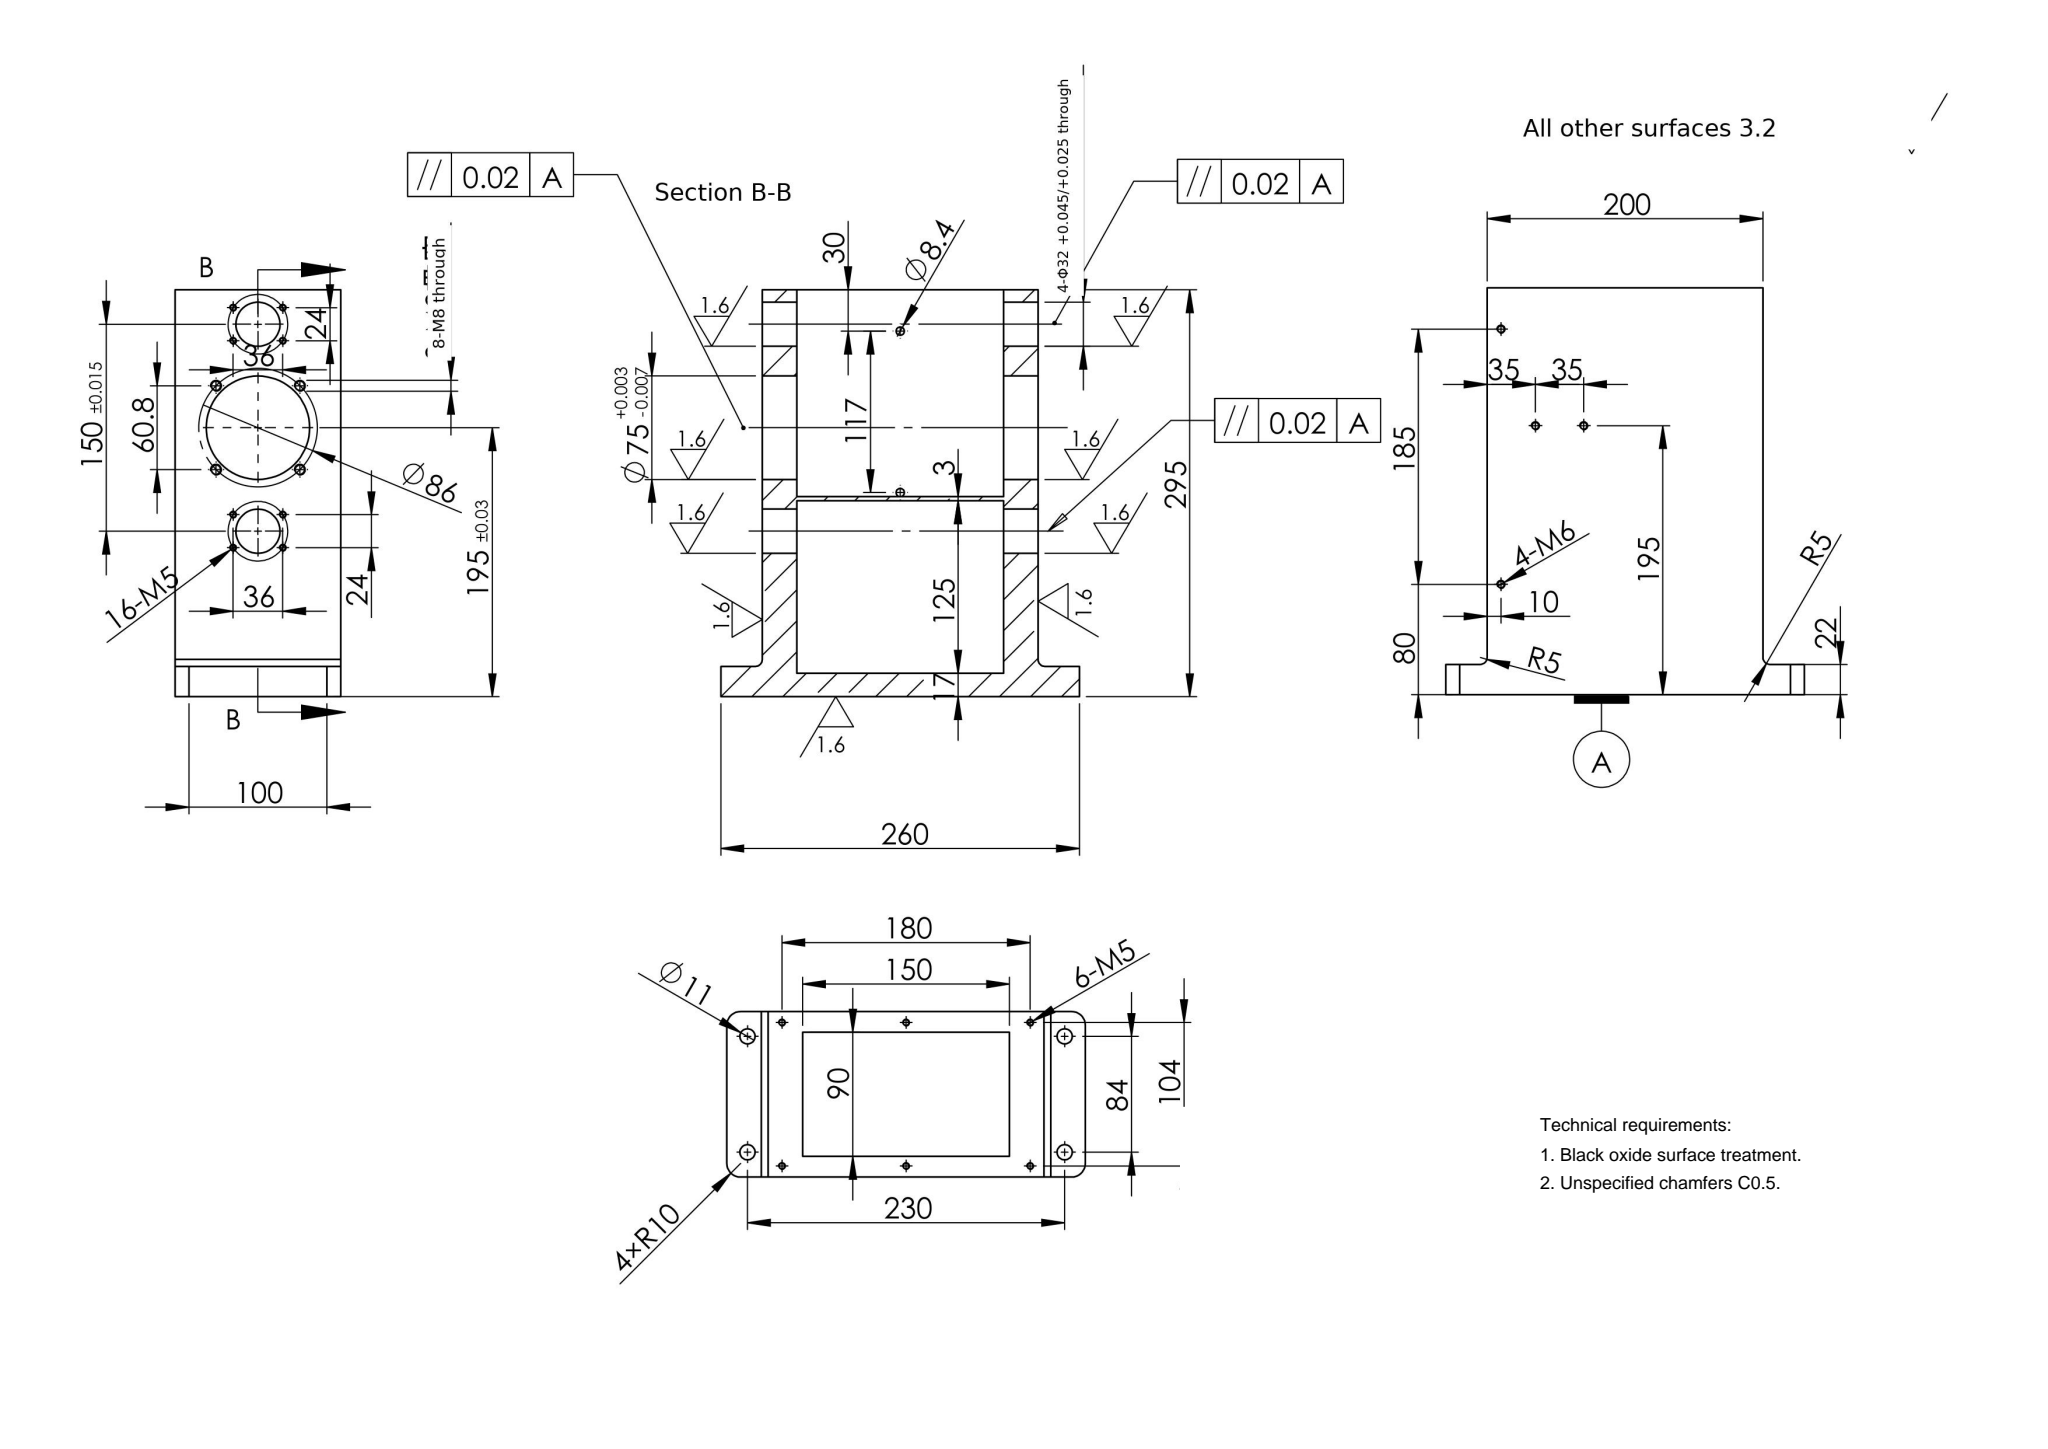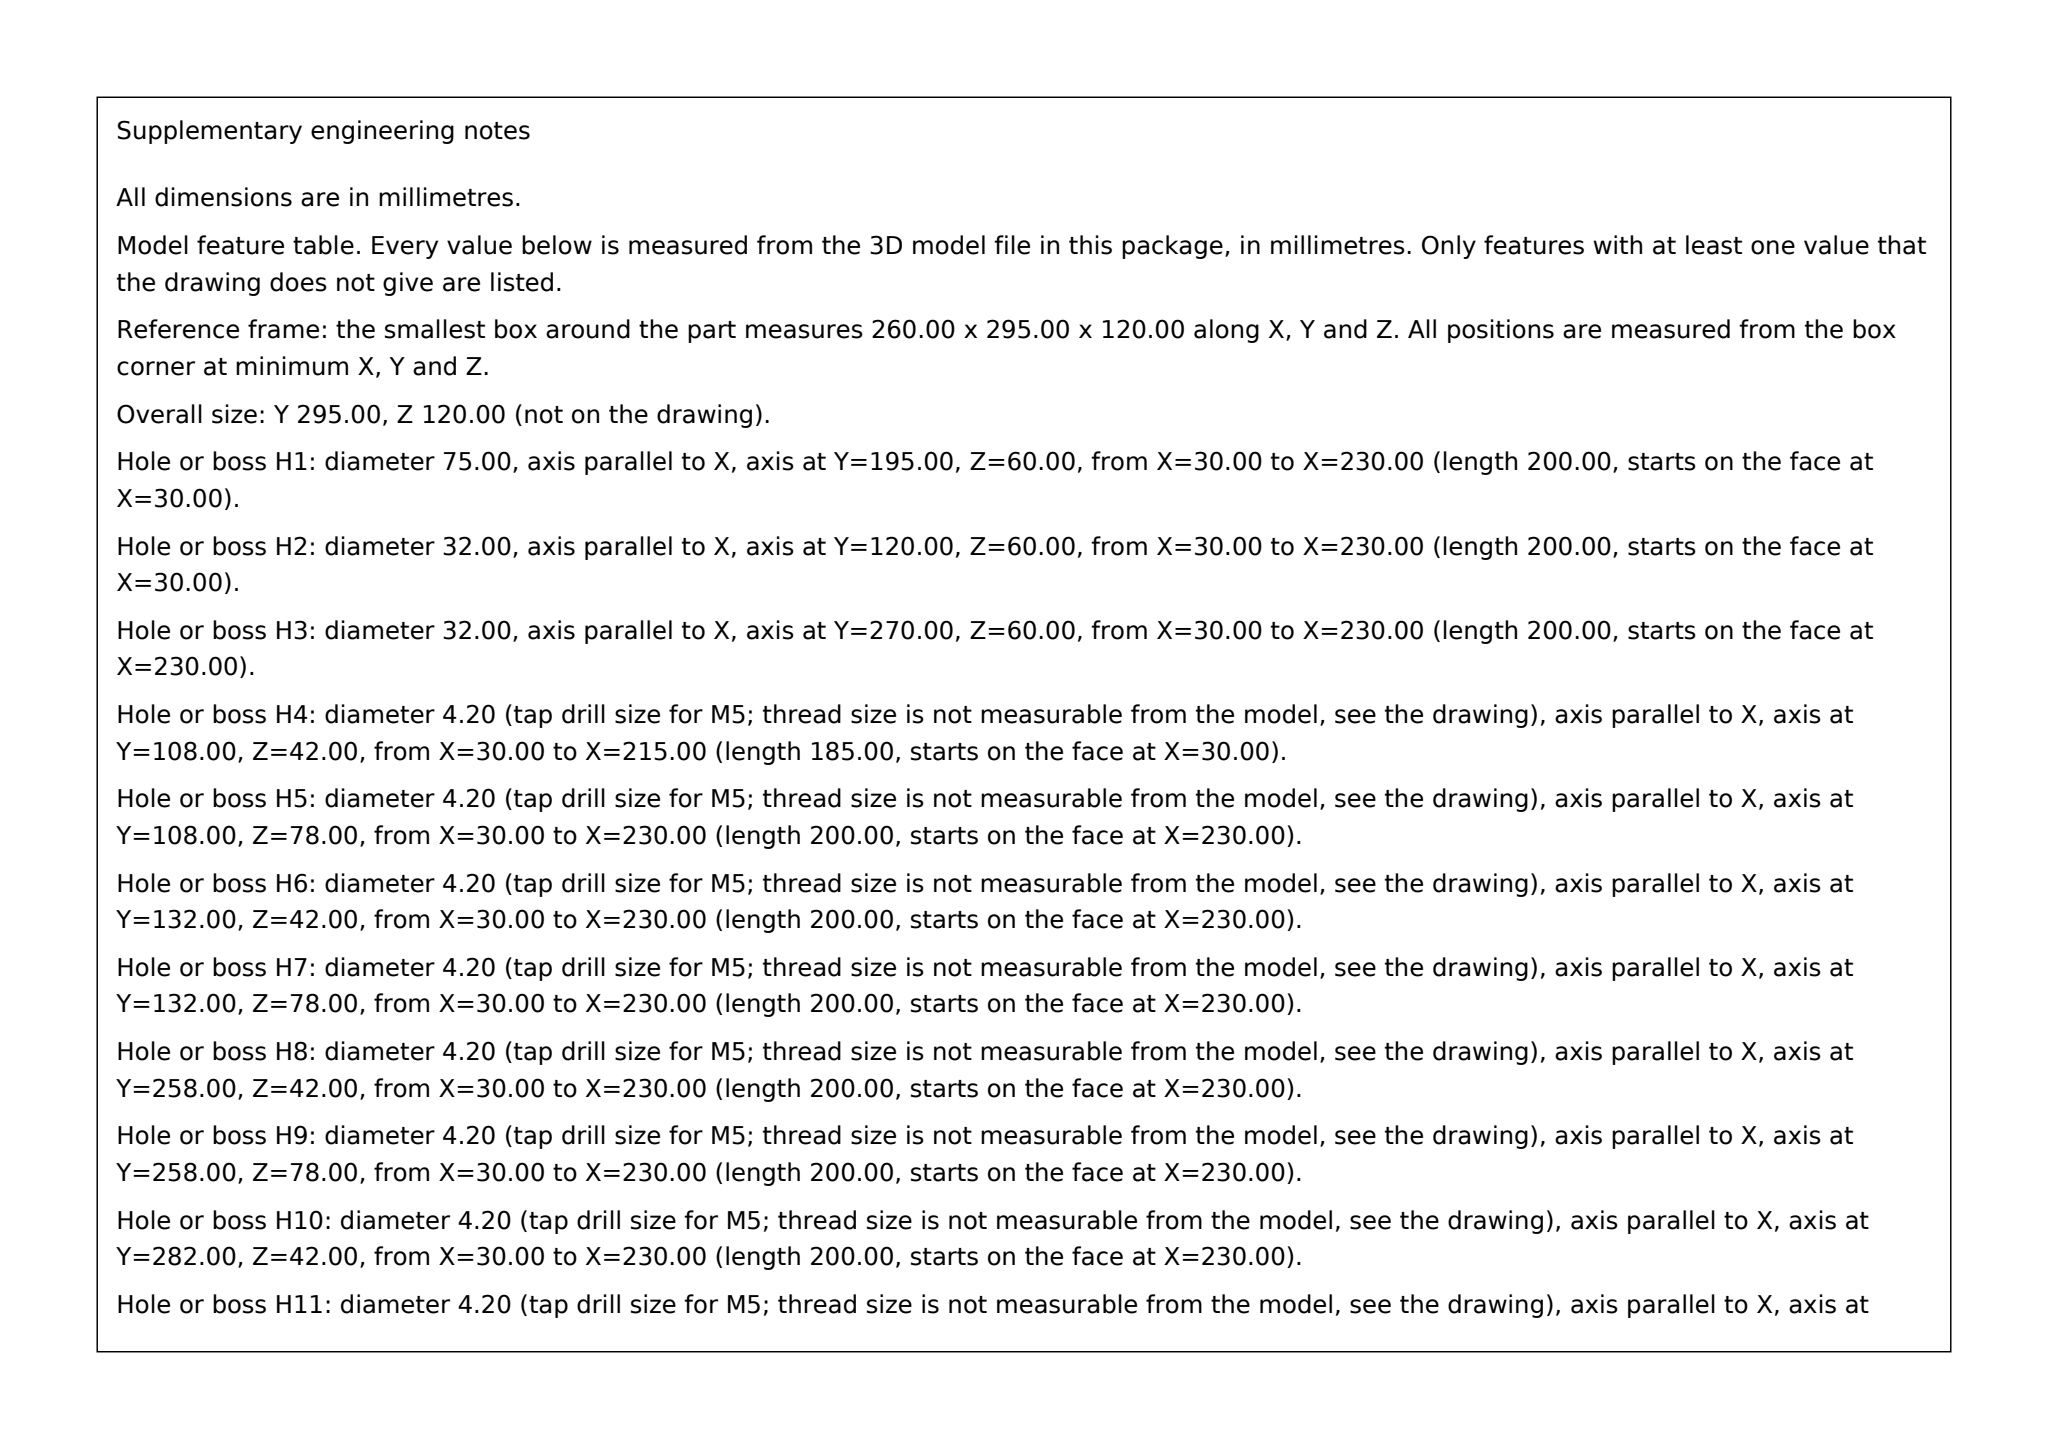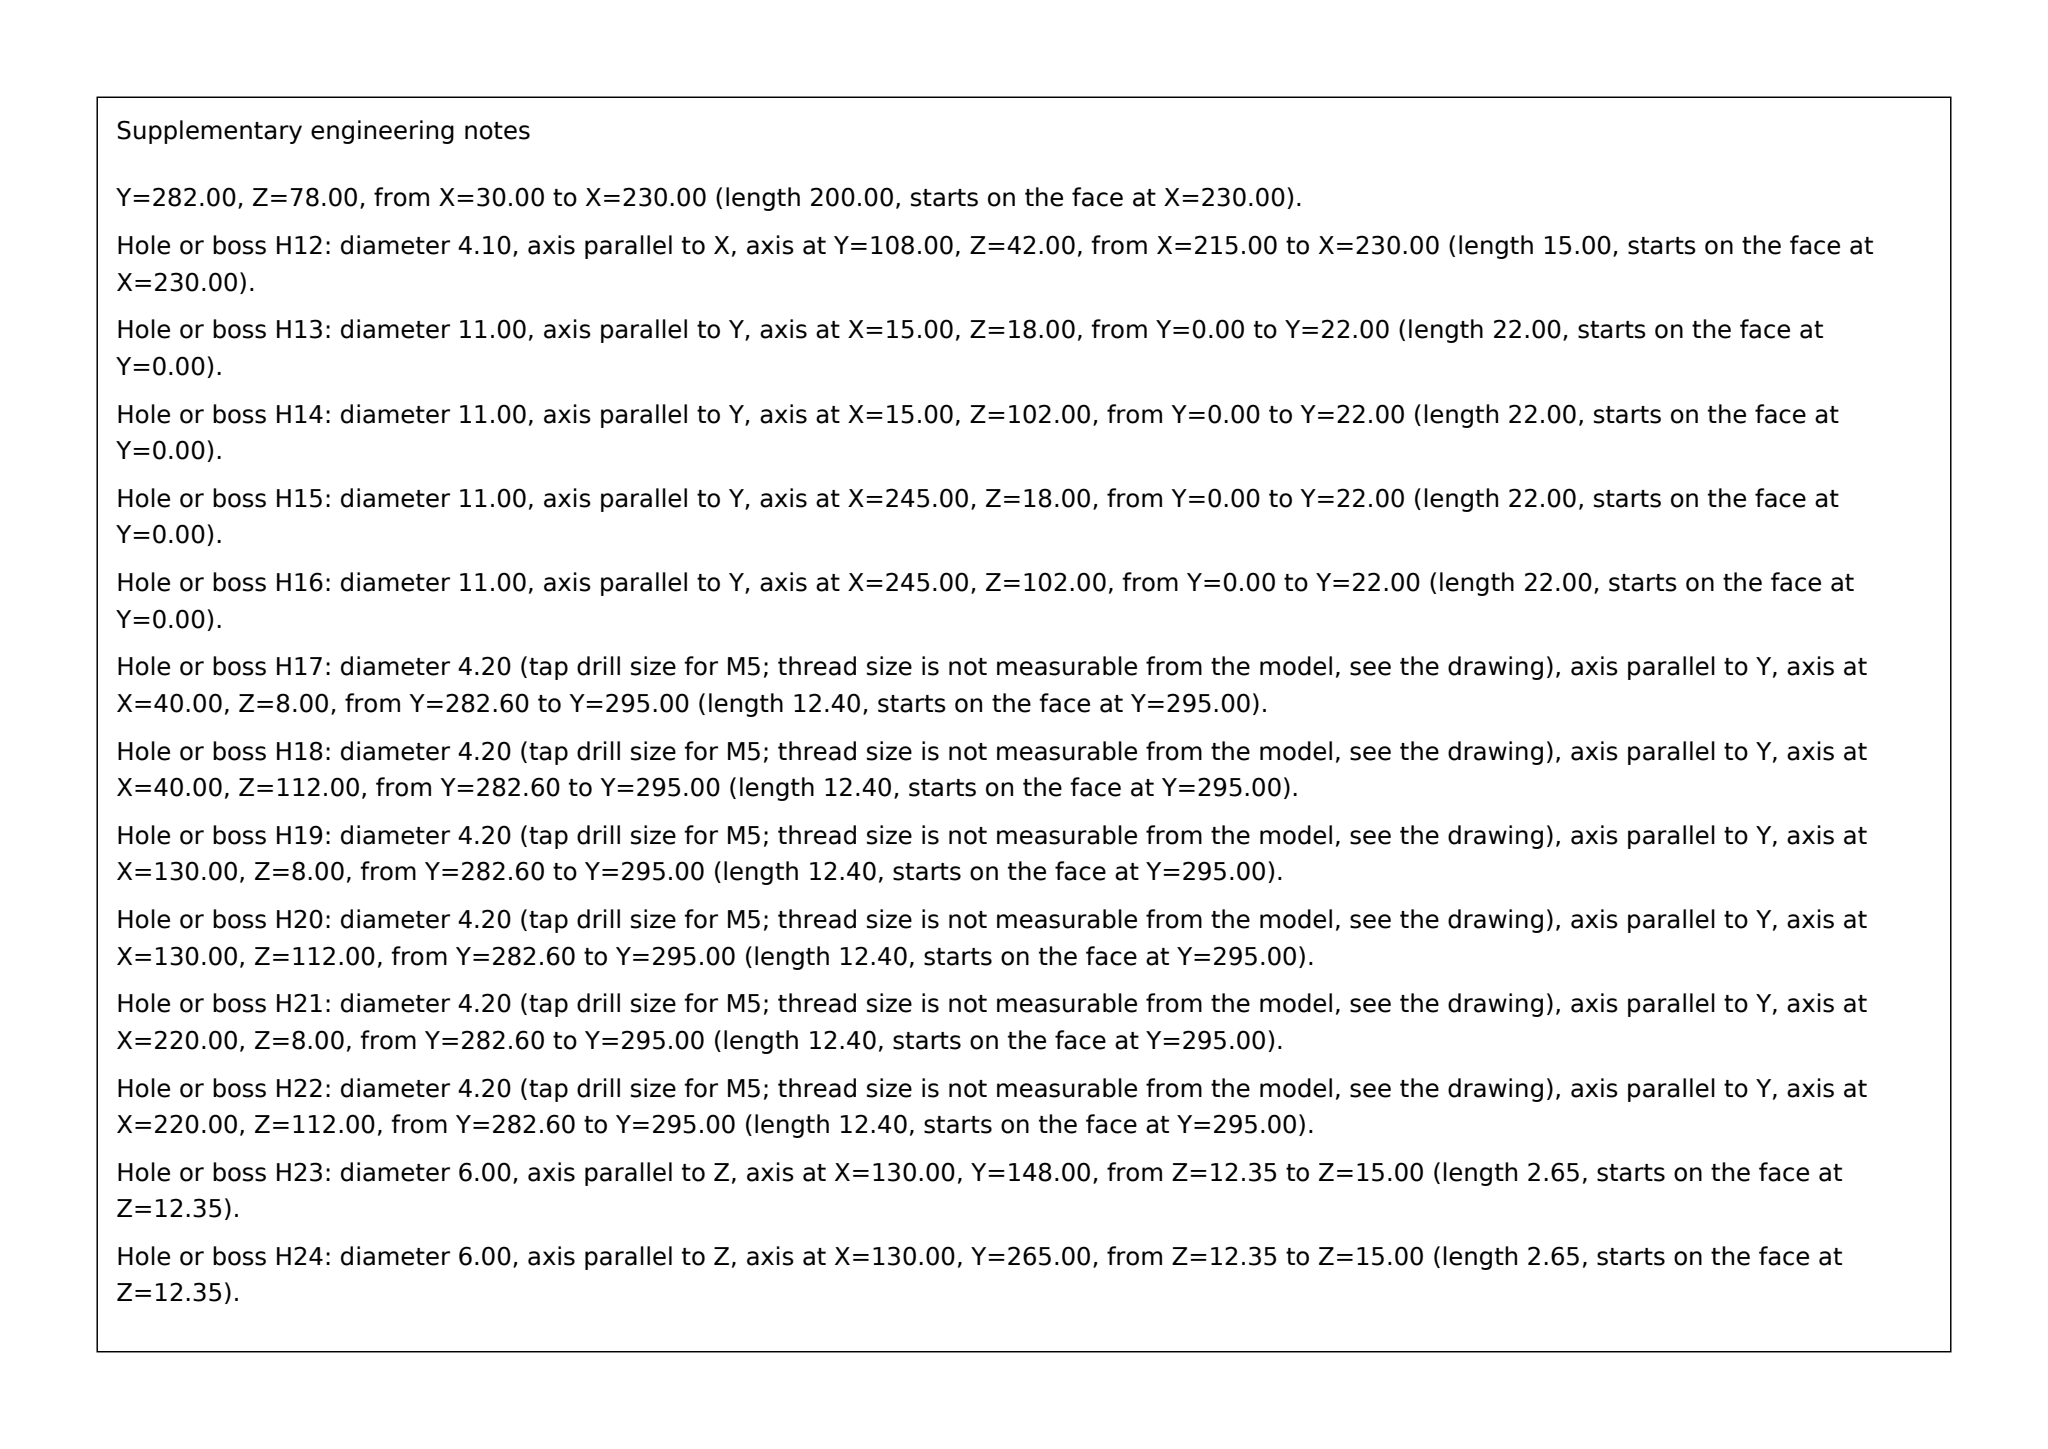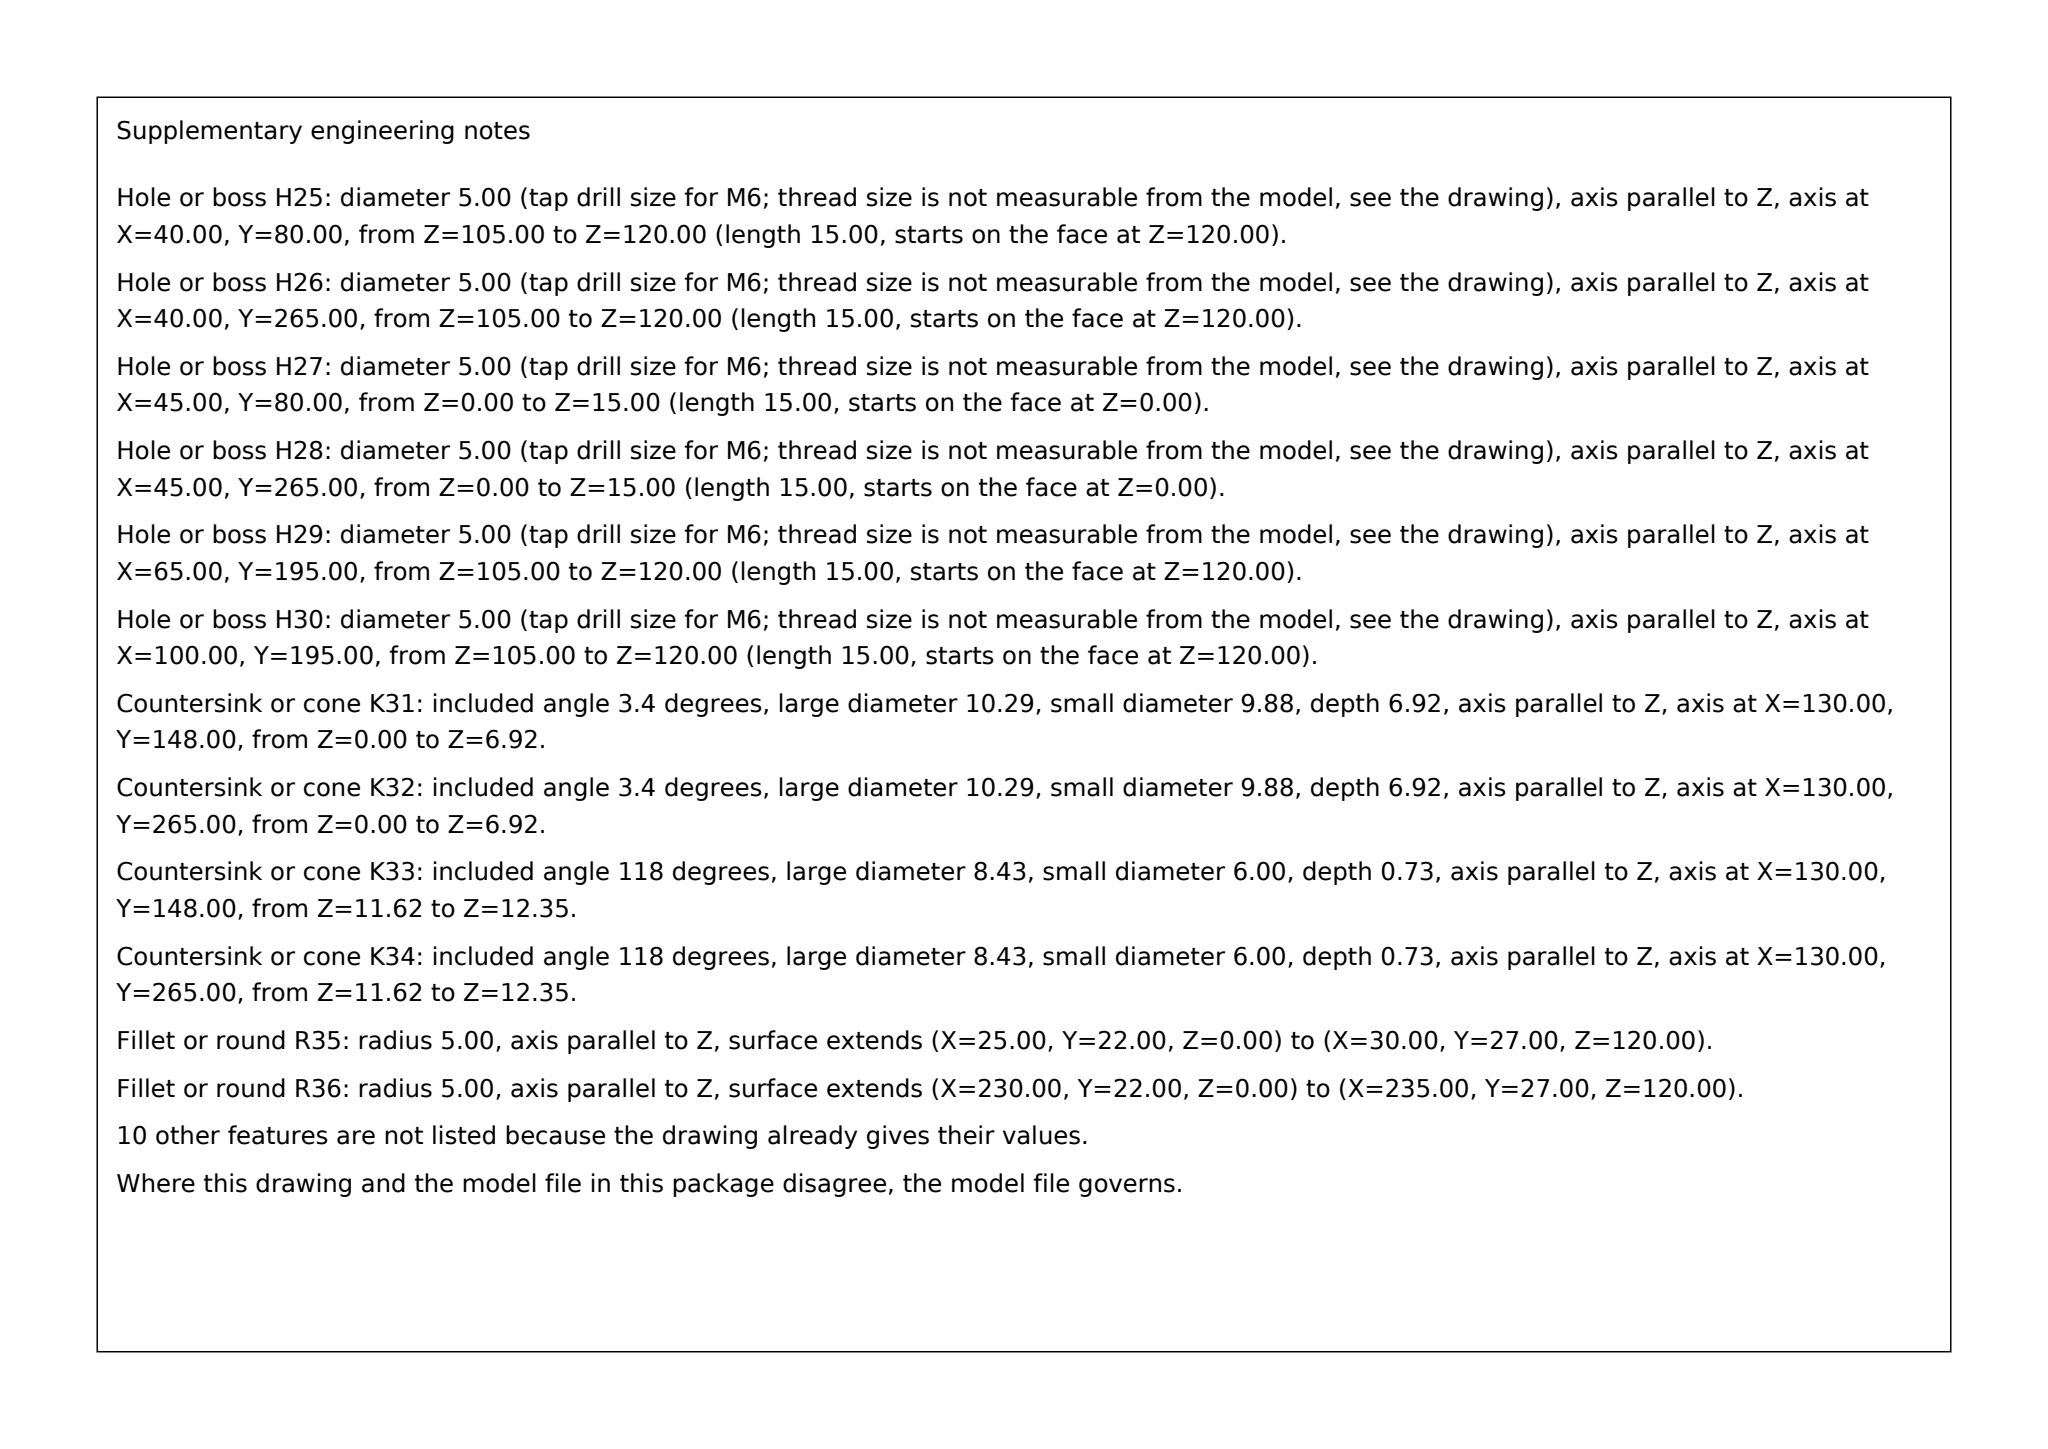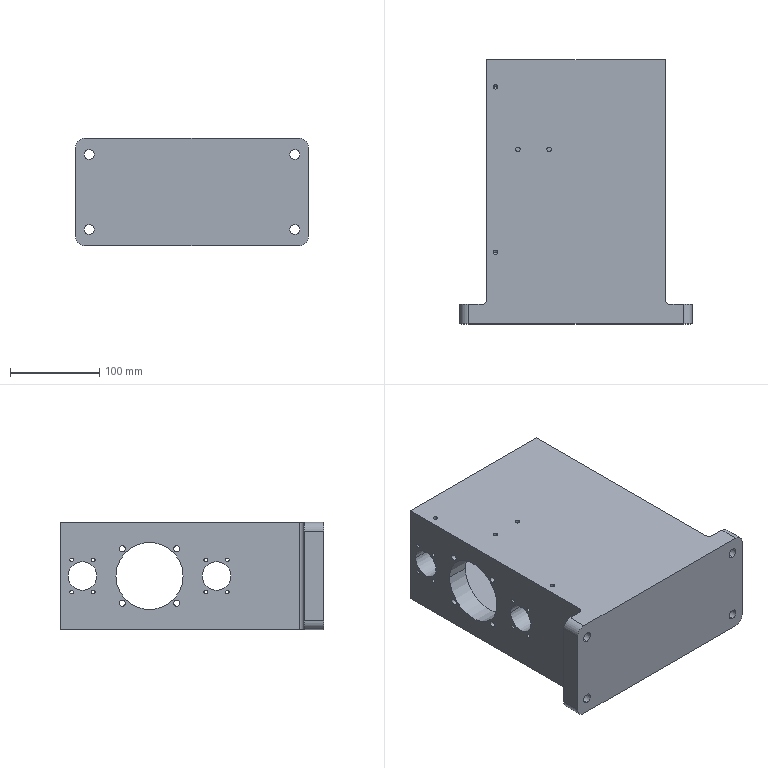Part | SolidWorks | mm | 1 solid | 160 faces | box 260 x 295 x 120 mm | volume 3198111 mm3 | cylinder 108 | cone 28 | plane 24 | commonest cylinder face diameters 4.2 x44 6.8 x16 5 x12 32 x8 11 x8 8.433 x4 6 x4 75 x4